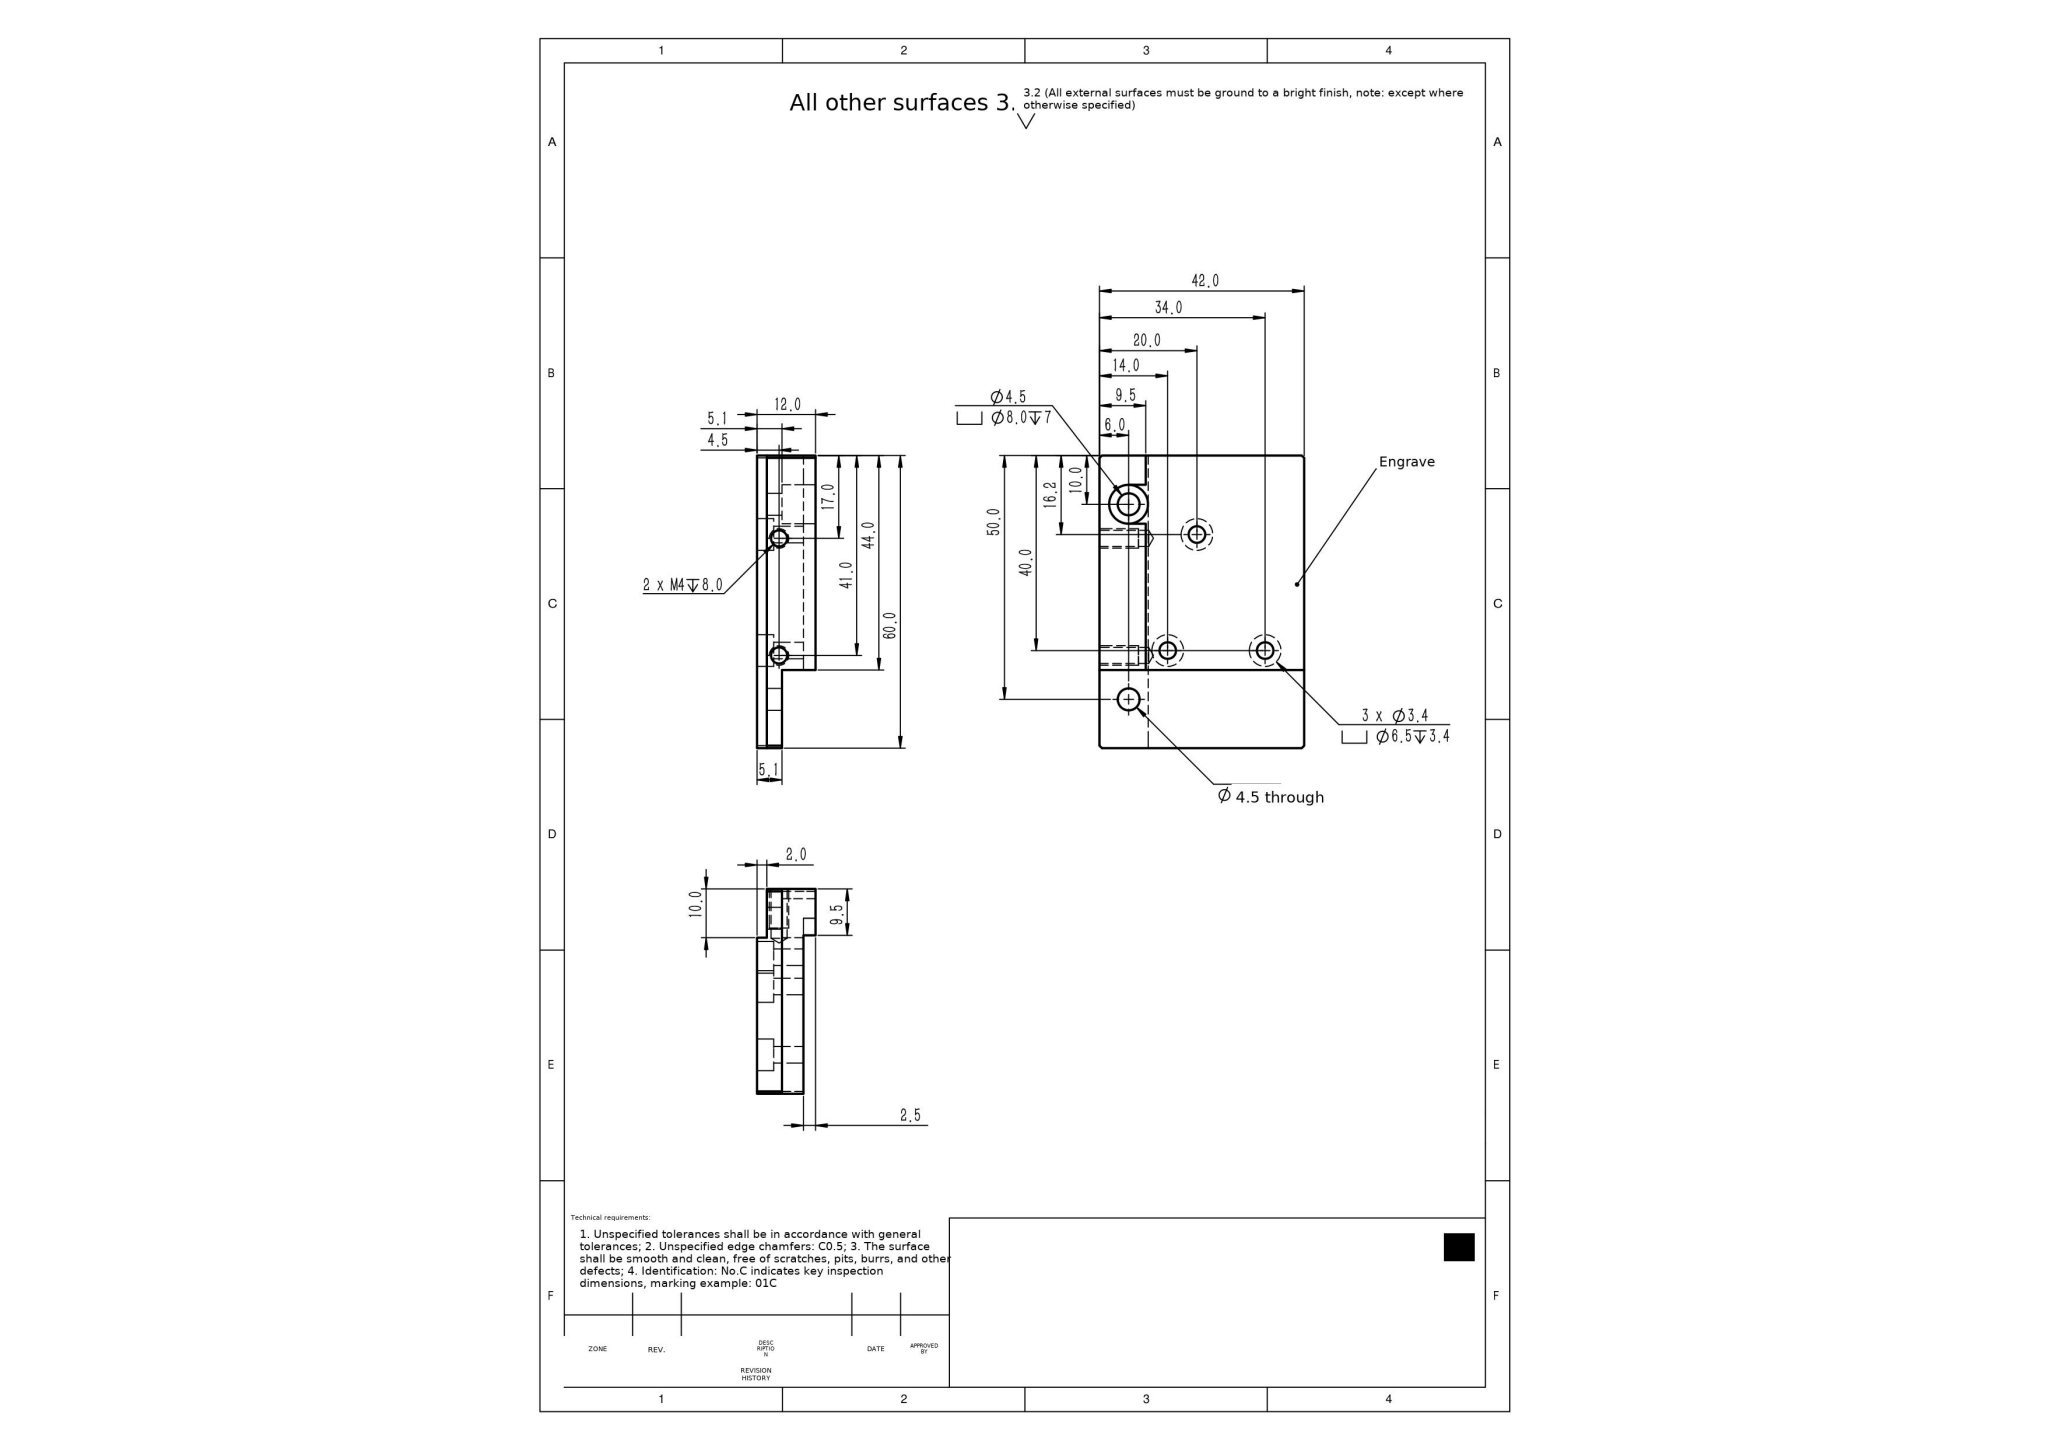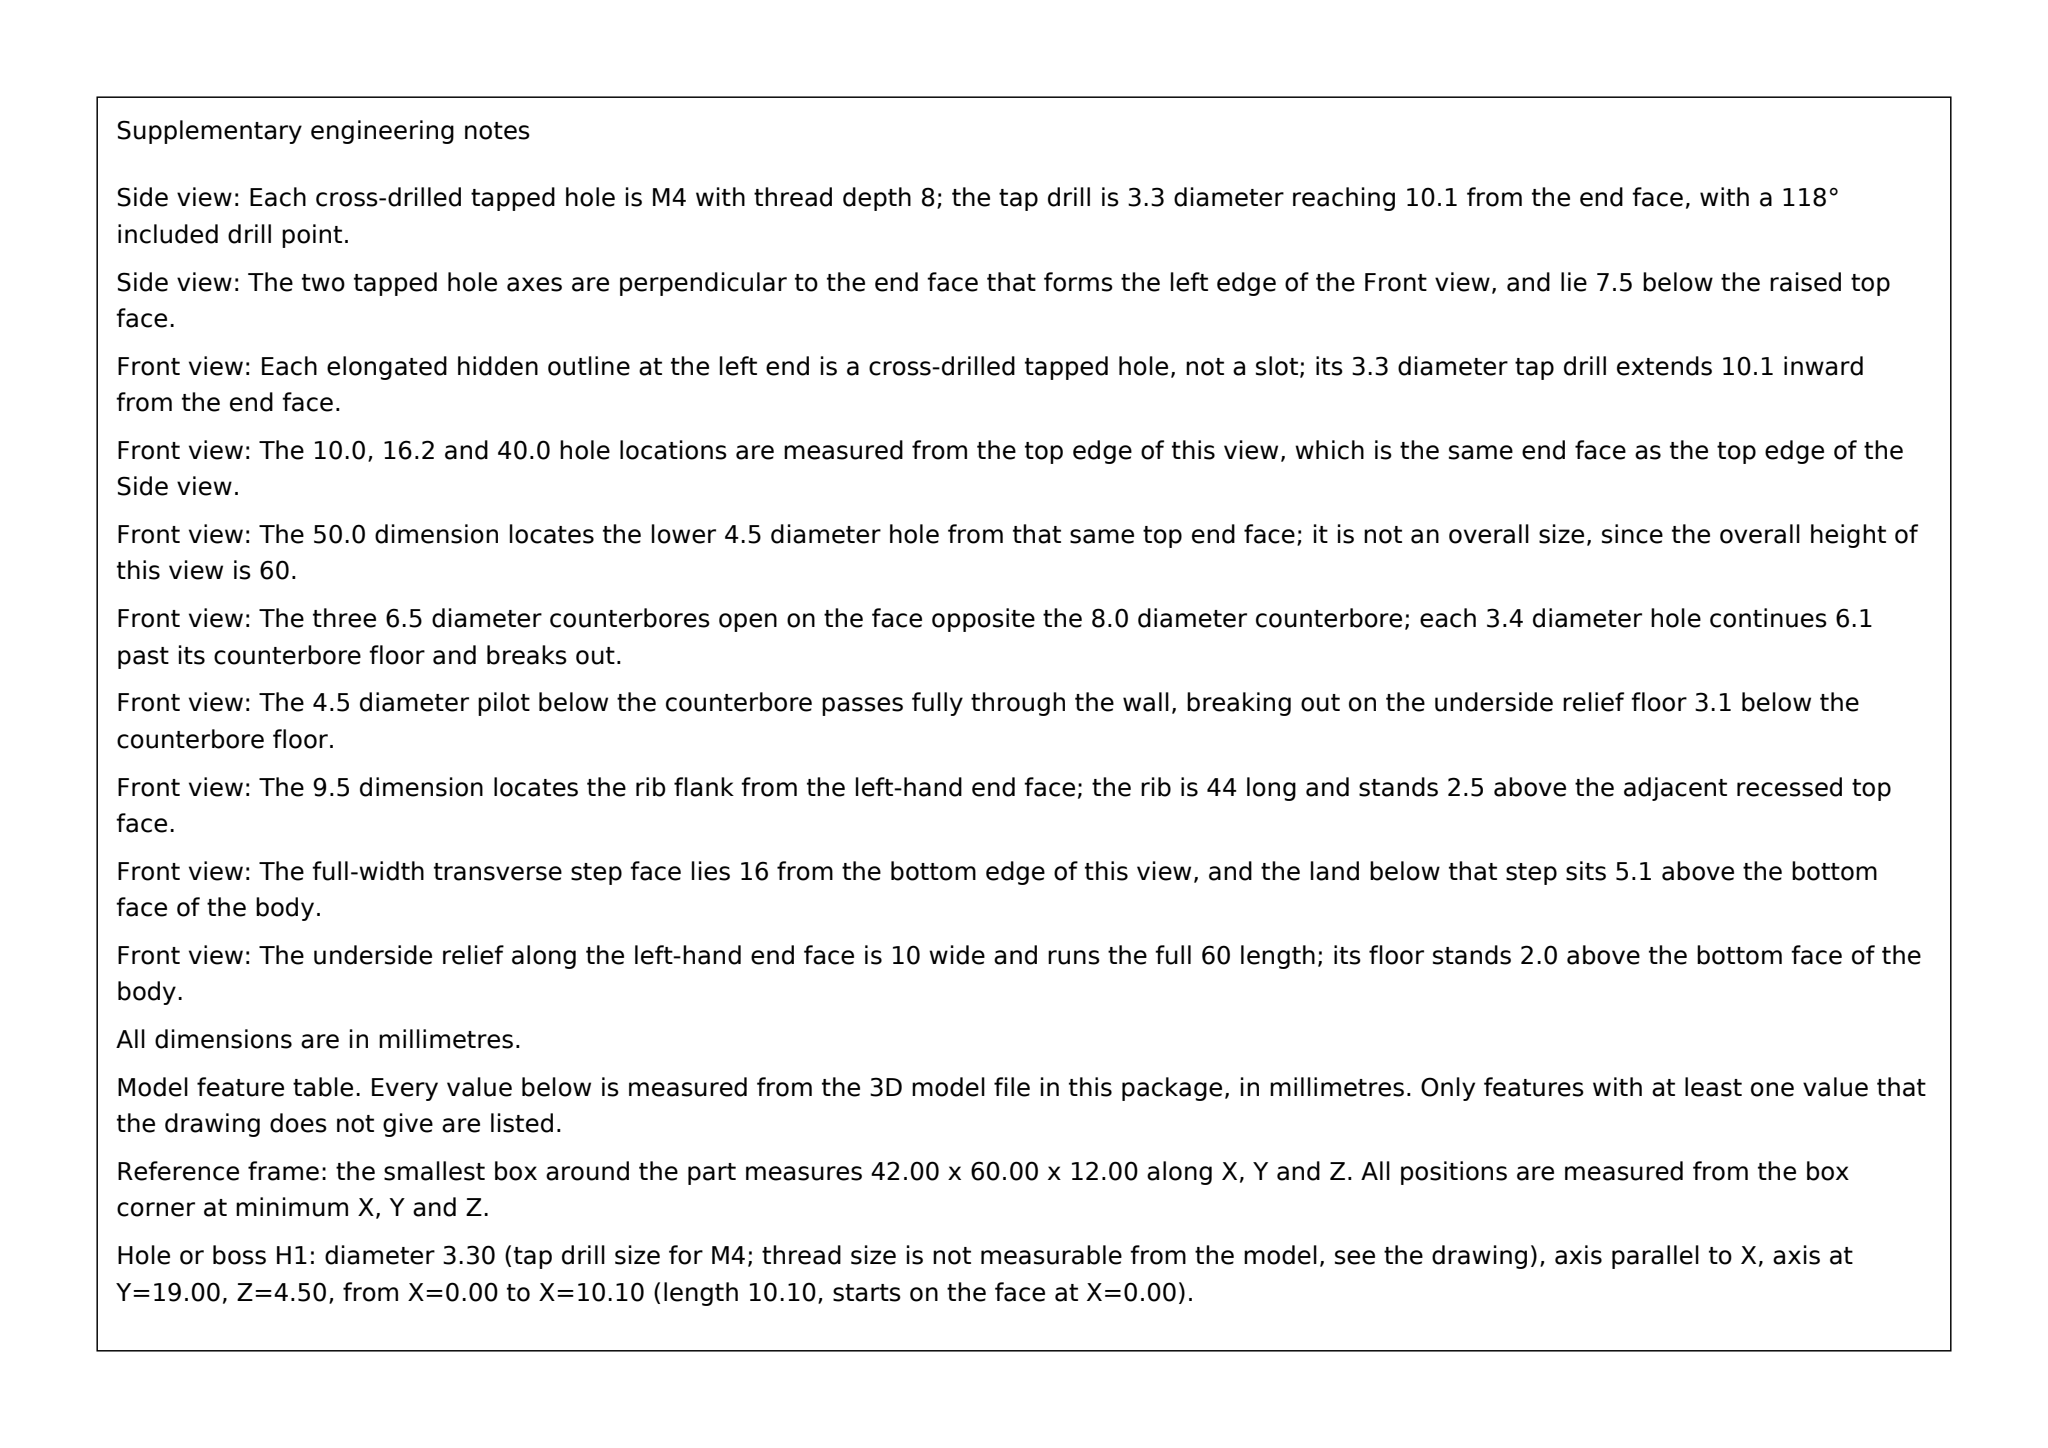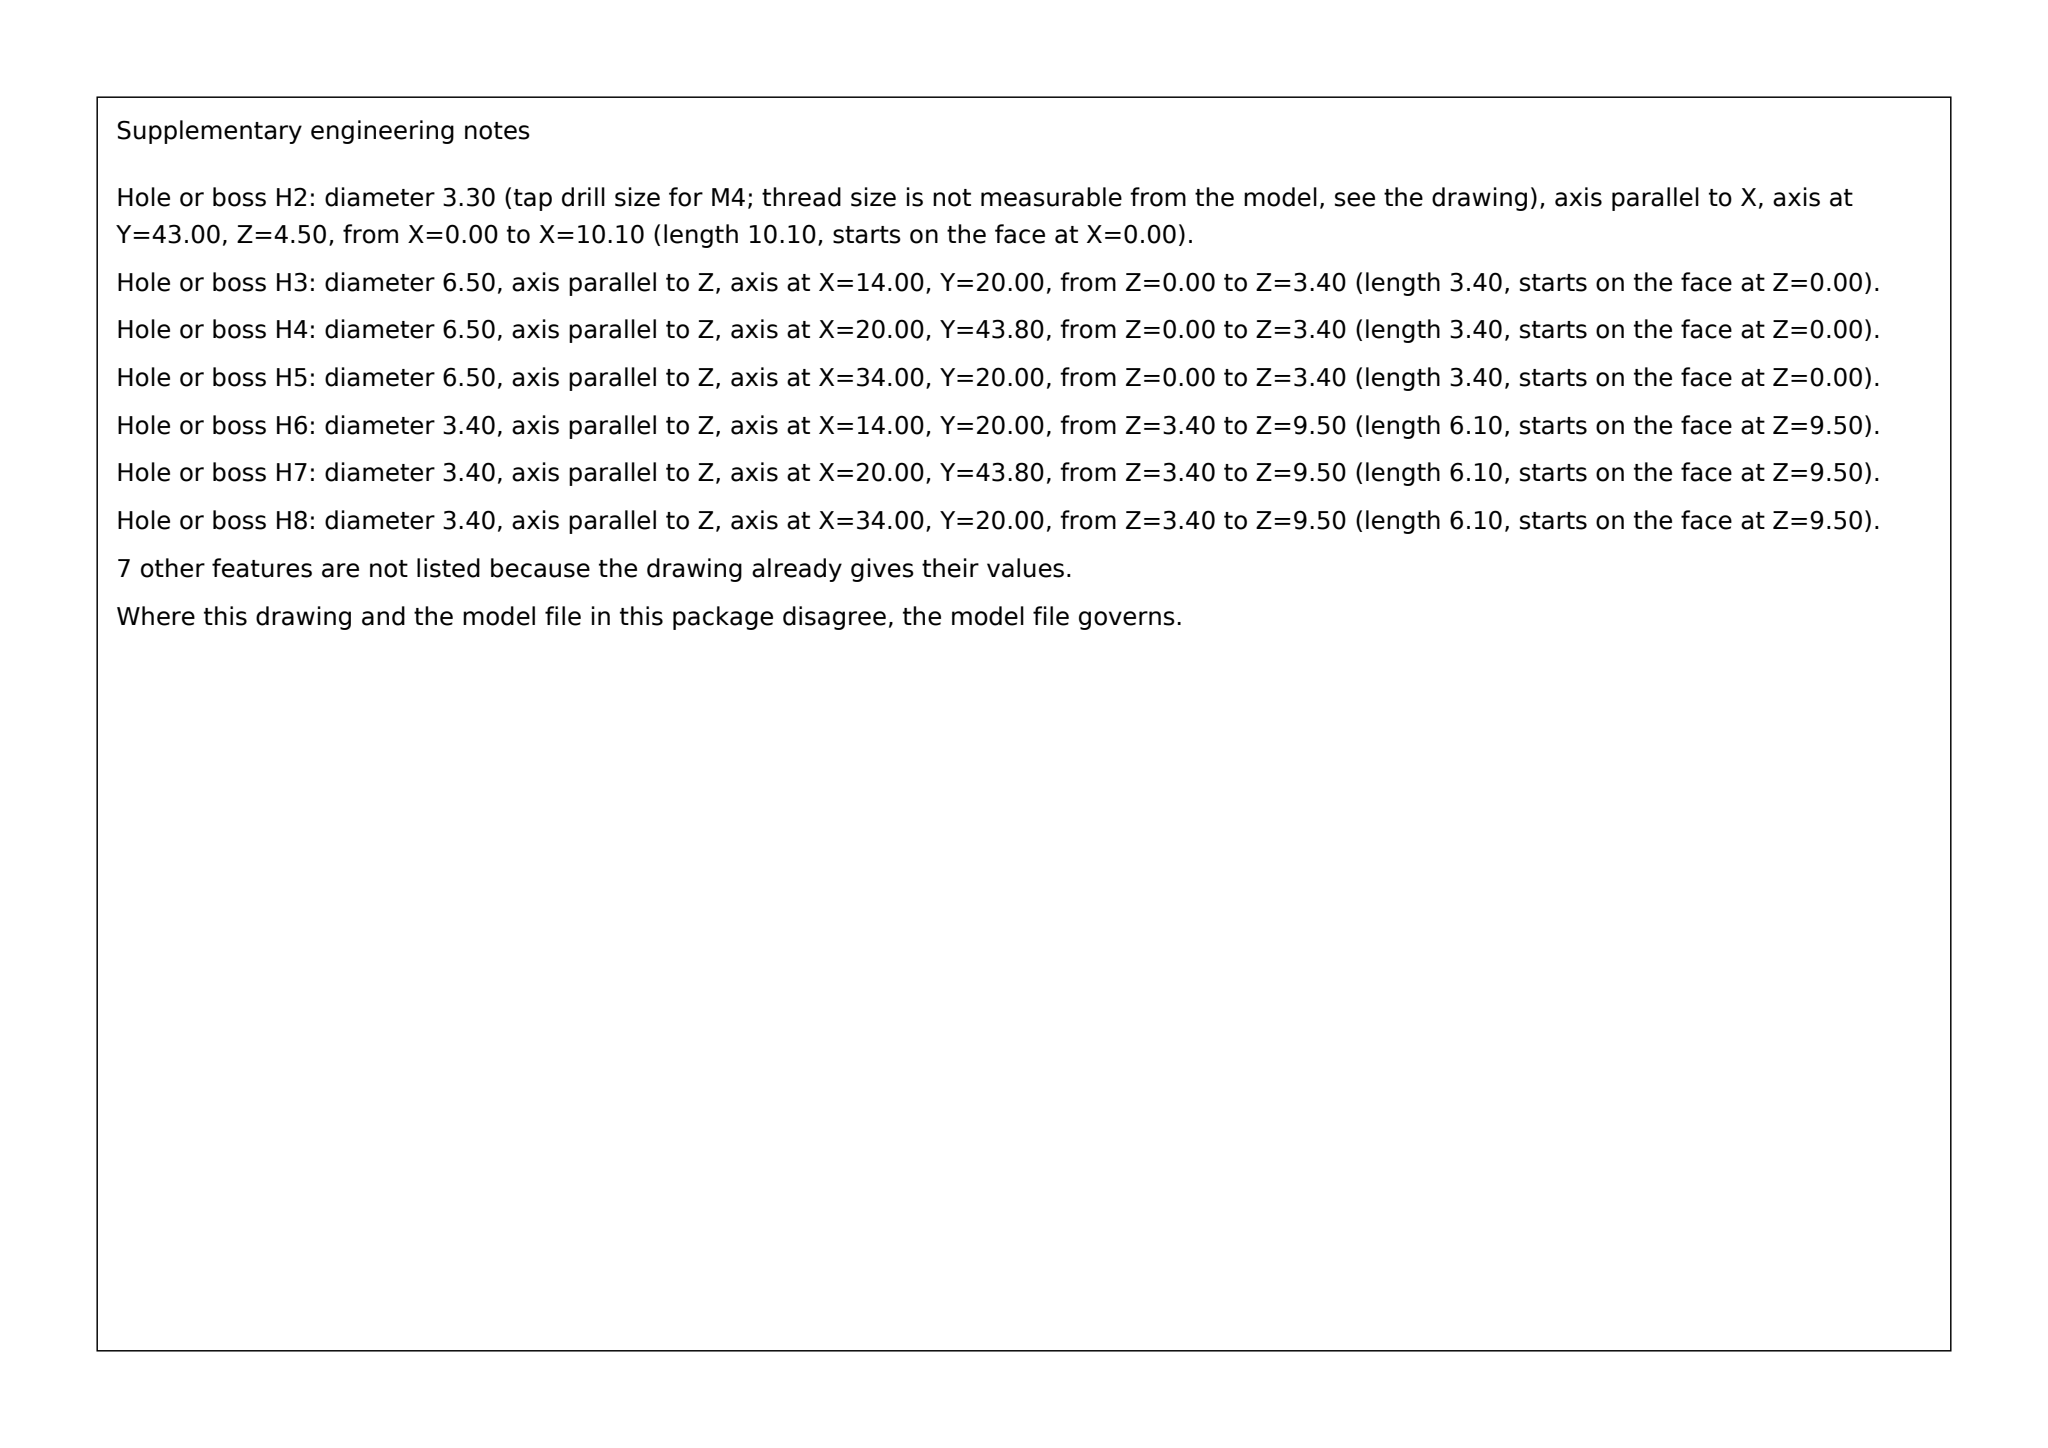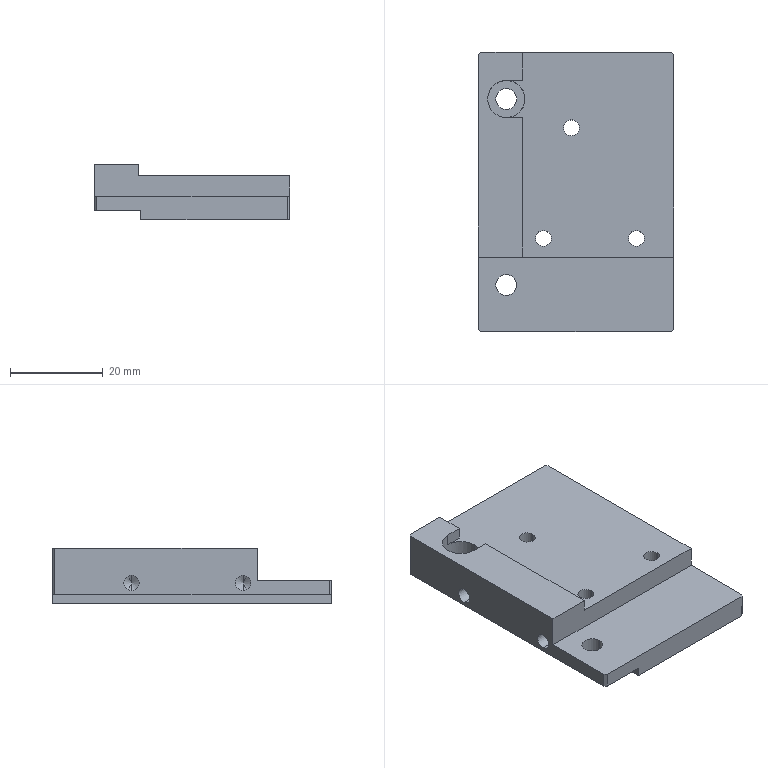Part | SolidWorks | mm | 1 solid | 49 faces | box 42 x 60 x 12 mm | volume 19689 mm3 | plane 23 | cylinder 22 | cone 4 | commonest cylinder face diameters 6.5 x6 3.4 x6 3.3 x4 4.5 x4 8 x2
Drawing notes:
OPEN SLOT IN TOP LAYER (Z 9.5 TO 12.0, DEPTH 2.5 FROM TOP FACE): 8.0 WIDE, SIDE FACES AT Y=46.0 AND Y=54.0 FROM BOTTOM EDGE (CENTRED ON Y=50.0), RUNNING FROM THE Ø8.0 CBORE AT X=6.0 AND OPEN AT THE STEP FACE X=9.5 FROM LEFT EDGE; NOT OPEN AT LEFT EDGE X=0 | from the solid: axis_planes: y=46.0 extent x[6.0,9.5] z[9.5,12.0] and y=54.0 extent x[6.0,9.5] z[9.5,12.0] (slot side faces, 8.0 apart, centred on Y=50.0); x=9.5 faces extent y[16.0,46.0] and y[54.0,60.0] z[9.5,12.0] (slot open through step face at X=9.5); z=9.5 face x[6.0,42.0] y[16.0,60.0] = slot floor; z=12.0 top face x[0.0,9.5] y[16.0,60.0]; x=0.0 face area 466 over y[0.5,59.5] z[2.0,12.0] is uninterrupted, so slot is not open at left edge; Ø8.0 bore at [6.0,50.0] from z 5.1 to 12.0
build123d program:
from build123d import *

# Parameters (mm, degrees)
SKETCH1_2_W                                     = 42
SKETCH1_2_H                                     = 60
BOSS_EXTRUDE1_DEPTH                             = 12
SKETCH3_W                                       = 40
SKETCH3_H                                       = 60
CUT_EXTRUDE1_DEPTH                              = 2.5
SKETCH6_W                                       = 10
SKETCH6_H                                       = 60
CUT_EXTRUDE2_DEPTH                              = 2
M4_HEX_SOCKET_HEAD_CAP_SCREW_CBORE1_D           = 4.5
M4_HEX_SOCKET_HEAD_CAP_SCREW_CBORE1_CBORE_D     = 8
M4_HEX_SOCKET_HEAD_CAP_SCREW_CBORE1_CBORE_DEPTH = 4.4
BOSS_EXTRUDE2_START                             = 2.5
BOSS_EXTRUDE2_DEPTH                             = 2.5
M3_HEX_SOCKET_HEAD_CAP_SCREW_CBORE1_D           = 3.4
M3_HEX_SOCKET_HEAD_CAP_SCREW_CBORE1_CBORE_D     = 6.5
M3_HEX_SOCKET_HEAD_CAP_SCREW_CBORE1_CBORE_DEPTH = 3.4
CHAMFER1_SIZE                                   = 0.5
SKETCH1_W                                       = 32.5
SKETCH1_H                                       = 16
EXTRUDE1_DEPTH                                  = 4.4
FILLET1_R                                       = 2
M4_TAPPED_HOLE1_D                               = 3.3
M4_TAPPED_HOLE1_DEPTH                           = 10.1
M4_TAPPED_HOLE1_TIP                             = 0.9914
SKETCH14_W                                      = 11.5
SKETCH14_H                                      = 16
CUT_EXTRUDE3_DEPTH                              = 6.9
SKETCH15_W                                      = 3.5
SKETCH15_H                                      = 8
CUT_EXTRUDE4_DEPTH                              = 2.5


with BuildPart() as part:
    # Sketch1_2 → Boss-Extrude1 (new body)
    with BuildSketch(Plane.XY):
        with Locations((21, 30)):
            Rectangle(SKETCH1_2_W, SKETCH1_2_H)
    extrude(amount=BOSS_EXTRUDE1_DEPTH)

    # Sketch3 → Cut-Extrude1 (cut)
    with BuildSketch(Plane.XY.offset(12)):
        with Locations((22, 30)):
            Rectangle(SKETCH3_W, SKETCH3_H)
    extrude(amount=-CUT_EXTRUDE1_DEPTH, mode=Mode.SUBTRACT)

    # Sketch6 → Cut-Extrude2 (cut)
    with BuildSketch(Plane(origin=(0, 0, 0), x_dir=(-1, 0, 0), z_dir=(0, 0, -1))):
        with Locations((-5, 30)):
            Rectangle(SKETCH6_W, SKETCH6_H)
    extrude(amount=-CUT_EXTRUDE2_DEPTH, mode=Mode.SUBTRACT)

    # M4 Hex Socket Head Cap Screw CBORE1 (through all)
    with Locations(Plane.XY.offset(9.5)):
        with Locations((6, 50), (6, 10)):
            CounterBoreHole(M4_HEX_SOCKET_HEAD_CAP_SCREW_CBORE1_D / 2, M4_HEX_SOCKET_HEAD_CAP_SCREW_CBORE1_CBORE_D / 2, M4_HEX_SOCKET_HEAD_CAP_SCREW_CBORE1_CBORE_DEPTH)

    # Sketch9 → Boss-Extrude2 (add)
    with BuildSketch(Plane.XY.offset(9.5).offset(BOSS_EXTRUDE2_START)):
        with BuildLine():
            Line((9.5, 60), (2, 60))
            Line((2, 60), (2, 50))
            ThreePointArc((2, 50), (5, 53.873), (9.5, 51.936))
            Line((9.5, 51.936), (9.5, 60))
        make_face()
        with BuildLine():
            ThreePointArc((9.5, 48.064), (5, 46.127), (2, 50))
            Line((2, 50), (2, 10))
            ThreePointArc((2, 10), (5, 13.873), (9.5, 11.936))
            Line((9.5, 11.936), (9.5, 48.064))
        make_face()
        with BuildLine():
            ThreePointArc((9.5, 8.064), (5, 6.127), (2, 10))
            Line((2, 10), (2, 0))
            Line((2, 0), (9.5, 0))
            Line((9.5, 0), (9.5, 8.064))
        make_face()
    extrude(amount=-BOSS_EXTRUDE2_DEPTH)

    # M3 Hex Socket Head Cap Screw CBORE1 (through all)
    with Locations(Plane(origin=(0, 0, 0), x_dir=(-1, 0, 0), z_dir=(0, 0, -1))):
        with Locations((-14, 20), (-34, 20), (-20, 43.8)):
            CounterBoreHole(M3_HEX_SOCKET_HEAD_CAP_SCREW_CBORE1_D / 2, M3_HEX_SOCKET_HEAD_CAP_SCREW_CBORE1_CBORE_D / 2, M3_HEX_SOCKET_HEAD_CAP_SCREW_CBORE1_CBORE_DEPTH)

    # Chamfer1
    chamfer1_edges = [part.edges().sort_by_distance(p)[0] for p in [
        (42, 60, 4.75),
        (42, 0, 4.75),
        (0, 60, 7),
        (0, 0, 7),
    ]]
    chamfer(chamfer1_edges, length=CHAMFER1_SIZE)

    # Sketch1 → Extrude1 (cut)
    with BuildSketch(Plane.XY.offset(9.5)):
        with Locations((25.75, 8)):
            Rectangle(SKETCH1_W, SKETCH1_H)
    extrude(amount=-EXTRUDE1_DEPTH, mode=Mode.SUBTRACT)

    # Fillet1
    fillet1_edges = [part.edges().sort_by_distance(p)[0] for p in [
        (9.5, 16, 7.3),
    ]]
    fillet(fillet1_edges, radius=FILLET1_R)

    # M4 Tapped Hole1
    with Locations(Plane.ZY):
        with Locations((4.5, 43), (4.5, 19)):
            Hole(M4_TAPPED_HOLE1_D / 2, depth=M4_TAPPED_HOLE1_DEPTH)
            with Locations((0, 0, -(M4_TAPPED_HOLE1_DEPTH + M4_TAPPED_HOLE1_TIP / 2))):  # 118° drill point
                Cone(0, M4_TAPPED_HOLE1_D / 2, M4_TAPPED_HOLE1_TIP, mode=Mode.SUBTRACT)

    # Sketch14 → Cut-Extrude3 (cut)
    with BuildSketch(Plane.XY.offset(12)):
        with Locations((5.75, 8)):
            Rectangle(SKETCH14_W, SKETCH14_H)
    extrude(amount=-CUT_EXTRUDE3_DEPTH, mode=Mode.SUBTRACT)

    # Sketch15 → Cut-Extrude4 (cut)
    with BuildSketch(Plane.XY.offset(12)):
        with Locations((7.75, 50)):
            Rectangle(SKETCH15_W, SKETCH15_H)
    extrude(amount=-CUT_EXTRUDE4_DEPTH, mode=Mode.SUBTRACT)


solid = part.part